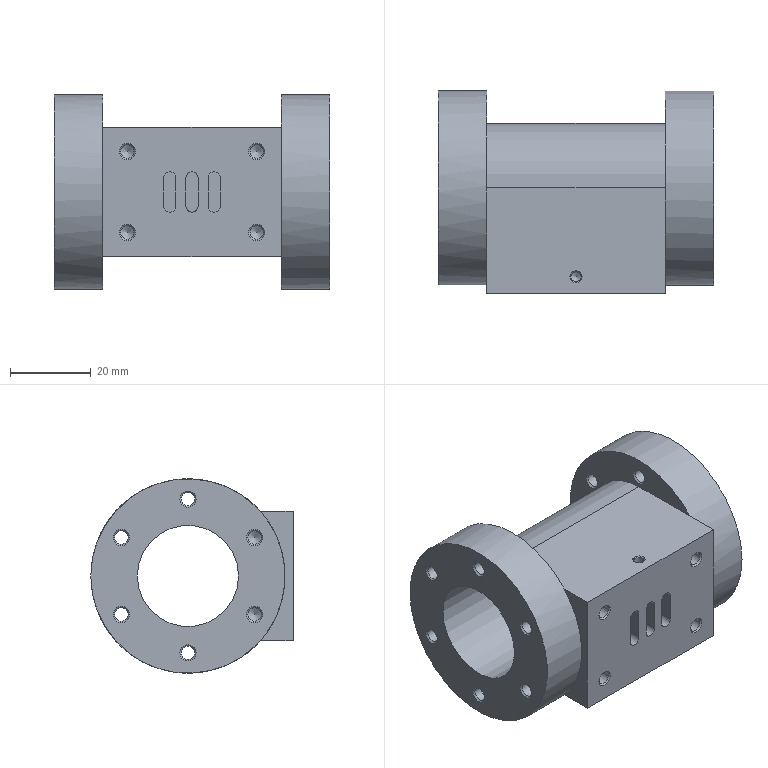Component | NX | PISTON_CYLINDER | 1 solid | 94 faces | volume 61215 mm3 | cone 40 | cylinder 33 | plane 21 | commonest cylinder face diameters 3.3 x16 3 x8 2.5 x3 48 x2 32 x1 25 x1 6.8 x1 5 x1